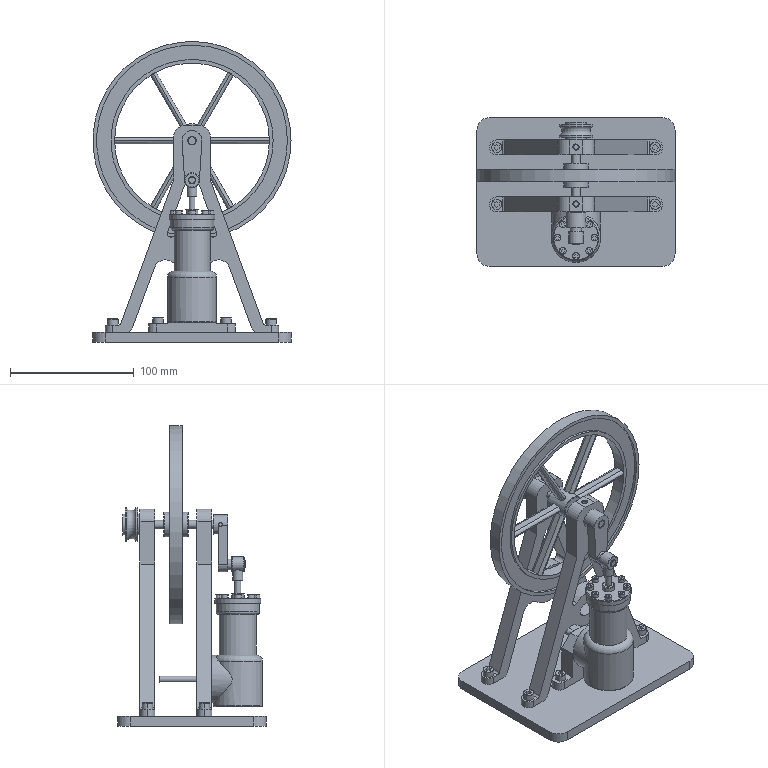Assembly | NX | mm | 29 component files | 29 solids | 591 faces | box 160 x 120 x 243 mm | volume 450330 mm3 | plane 256 | cylinder 219 | torus 67 | cone 49 | commonest cylinder face diameters 5 x50 3 x28 5.5 x20 12 x18 8.5 x12 20 x9 4 x8 3.4 x8
Bill of materials:
unnamed part 1 | 1 |  | Short solid-of-revolution disc with a small central through-hole and one shallow rectangular circumferential groove around the outside, making a spool-like profile.
unnamed part 2 | 2 |  | Flat, symmetric A-shaped bracket plate. It has a rounded top tab with a hole, two diverging legs ending in small flat feet with holes, and a central ring with an oval through-opening joining the legs.
unnamed part 3 | 1 |  | Round flange disc with a central hub boss on one face, a shorter wide spigot on the other face, a central through-bore, and eight through-holes equally spaced on a bolt circle.
unnamed part 4 | 1 |  | T-shaped tubular fitting: a short thick-walled cylindrical sleeve with a through-bore, joined at right angles to a solid cylindrical stem.
unnamed part 5 | 1 |  | Long straight cylindrical rod with a small cross pin passing through it near one end, sticking out both sides.
unnamed part 6 | 1 |  | Stepped cylindrical housing or tee body: a larger lower cylinder, a smaller upper tubular neck ending in a flange with a bore and eight small holes on a bolt circle, and a cylindrical side branch on the lower body.
unnamed part 7 | 1 |  | Plain solid cylindrical rod with flat ends and no visible features.
unnamed part 8 | 1 |  | Tapered crank-arm lever: a flat link with a rounded wide end holding a through-bore inside a thicker boss, and a narrower rounded end carrying a stepped cylindrical pin that projects perpendicular to the arm.
unnamed part 9 | 6 |  | Socket-head cap-screw-like fastener shape: a cylindrical head with a hexagonal socket recess, and a plain cylindrical shank with a chamfered tip.
unnamed part 10 | 1 |  | Long slender cylindrical pin or shaft with a short reduced-diameter step at one end.
unnamed part 11 | 8 |  | Socket-head cap-screw-like fastener shape: a cylindrical head with a hexagonal socket and a plain cylindrical shank with a chamfered end. Its proportions are similar to the other cap-screw-like part.
unnamed part 12 | 1 |  | Grooved wheel or sheave: a solid of revolution with a central through-bore, a deep concave (U/V-radiused) circumferential groove between two flanges, and short hub bosses projecting from both faces.
unnamed part 13 | 1 |  | Thin flat rectangular plate with rounded corners and six small round through-holes: two near one long edge, and four in a row along the opposite side (two near the corners, two further inboard).
unnamed part 14 | 1 |  | Thin-walled cylindrical split ring (open band) with a single narrow angled gap cut through the wall.
unnamed part 15 | 1 |  | Spoked wheel: a wide flat outer rim joined to a central cylindrical hub by six thin round spokes evenly spaced at 60 degrees. The hub has a small central bore and sticks out axially on both sides of the rim.
unnamed part 16 | 1 |  | Upright bracket: a vertical rectangular block with both top corners chamfered, sitting on a narrow base flange with rounded ends. Each end of the flange has one counterbored or chamfered through-hole. The upright face has one larger hole near the top and two smaller holes side by side below it, all going through.
Mates:
1. fix | Base 1 component
2. concentric | Bracket 2 edge | Base 1 edge
3. concentric | Bracket 2 edge | Base 1 edge
4. concentric | Bracket 1 edge | Base 1 edge
5. concentric | Bracket 1 edge | Base 1 edge
6. concentric | Support_Frame 1 edge | Base 1 edge
7. parallel | Support_Frame 1 face | Base 1 face
8. touch align | Flywheel 1 face | Bracket 1 face
9. center | Flywheel 1 face | Flywheel 1 face | Bracket 2 face | Bracket 1 face
10. touch align | Flywheel_Shaft 1 face | Bracket 1 face
11. center | Flywheel_Shaft 1 face | Flywheel_Shaft 1 face | Bracket 2 face | Bracket 1 face
12. touch align | Cam 1 face | Flywheel_Shaft 1 face
13. touch align | Cam 1 face | Flywheel_Shaft 1 face
14. touch align | Pulley 1 face | Flywheel_Shaft 1 face
15. touch align | Pulley 1 face | Bracket 2 face
16. concentric | Cylinder_Head 1 edge | Cylinder 1 arc
17. concentric | Cylinder_Head 1 edge | Cylinder 1 edge
18. concentric | Cylinder 1 edge | Support_Frame 1 edge
19. concentric | Cylinder_Shaft 1 edge | Cylinder 1 edge
20. concentric | Piston_Ring 1 arc | Piston 1 edge
21. concentric | Piston_Rod 1 edge | Piston 1 arc
22. concentric | Piston_Rod 1 edge | Piston_Link 1 edge
23. touch align | Piston_Rod 1 face | Cylinder_Head 1 face
24. touch align | Piston_Link 1 face | Cam 1 face
25. concentric | Hex_Screw_M5x12 6 edge | Bracket 1 edge
26. concentric | Hex_Screw_M5x12 5 edge | Bracket 2 edge
27. concentric | Hex_Screw_M5x12 4 edge | Bracket 2 edge
28. concentric | Hex_Screw_M5x12 3 edge | Bracket 1 edge
29. concentric | Hex_Screw_M5x12 2 edge | Support_Frame 1 edge
30. concentric | Hex_Screw_M5x12 1 edge | Support_Frame 1 edge
31. concentric | Hex_Screw_M3x10 8 edge | Cylinder_Head 1 edge
32. bond | Cylinder_Head 1 component | assembly component
33. bond | Hex_Screw_M3x10 8 component | assembly component
34. bond | Hex_Screw_M3x10 7 component | assembly component
35. bond | Hex_Screw_M3x10 6 component | assembly component
36. bond | Hex_Screw_M3x10 5 component | assembly component
37. circular | assembly datumaxis | assembly cartesiancoordinatesystem | assembly cartesiancoordinatesystem | assembly cartesiancoordinatesystem | assembly cartesiancoordinatesystem | assembly cartesiancoordinatesystem | assembly cartesiancoordinatesystem | assembly cartesiancoordinatesystem | assembly cartesiancoordinatesystem
38. bond | Hex_Screw_M3x10 4 component | assembly component
39. bond | Hex_Screw_M3x10 3 component | assembly component
40. bond | Hex_Screw_M3x10 2 component | assembly component
41. bond | Hex_Screw_M3x10 1 component | assembly component